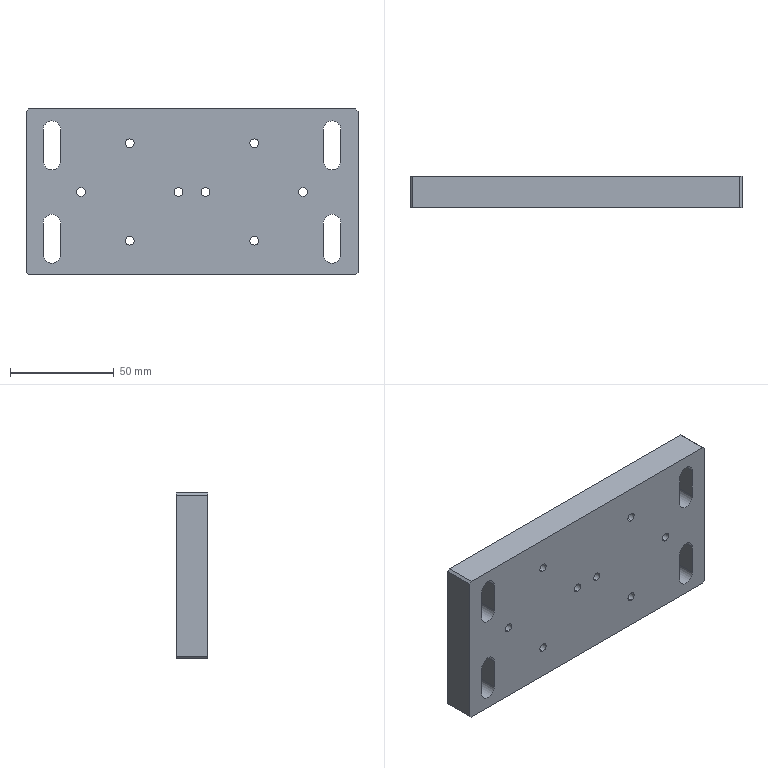Component | SolidWorks | CCDJSBottomFixingPlate-1 | 1 solid | 46 faces | box 160 x 15 x 80 mm | volume 179253 mm3 | cylinder 28 | plane 18 | commonest cylinder face diameters 4.2 x16 8.5 x12 | material 45#
build123d program:
from build123d import *

# Parameters (mm, degrees)
SKETCH1_W           = 160
SKETCH1_H           = 80
BOSS_EXTRUDE1_DEPTH = 15
CHAMFER1_SIZE       = 1
CUT_EXTRUDE1_DEPTH  = 32
M5_TAPPED_HOLE1_D   = 4.2


with BuildPart() as part:
    # Sketch1 → Boss-Extrude1 (new body)
    with BuildSketch(Plane(origin=(0, 0, 0), x_dir=(1, 0, 0), z_dir=(0, 1, 0))):
        Rectangle(SKETCH1_W, SKETCH1_H)
    extrude(amount=BOSS_EXTRUDE1_DEPTH)

    # Chamfer1
    chamfer1_edges = [part.edges().sort_by_distance(p)[0] for p in [
        (80, 7.5, 40),
        (-80, 7.5, 40),
        (-80, 7.5, -40),
        (80, 7.5, -40),
    ]]
    chamfer(chamfer1_edges, length=CHAMFER1_SIZE)

    # Sketch2 → Cut-Extrude1 (cut)
    with BuildSketch(Plane(origin=(0, 15, 0), x_dir=(1, 0, 0), z_dir=(0, 1, 0))):
        with BuildLine():
            Line((-63.25, 30), (-63.25, 15))
            ThreePointArc((-63.25, 15), (-67.5, 10.75), (-71.75, 15))
            Line((-71.75, 15), (-71.75, 30))
            ThreePointArc((-71.75, 30), (-67.5, 34.25), (-63.25, 30))
        make_face()
        with BuildLine():
            Line((-63.25, -30), (-63.25, -15))
            ThreePointArc((-63.25, -15), (-67.5, -10.75), (-71.75, -15))
            Line((-71.75, -15), (-71.75, -30))
            ThreePointArc((-71.75, -30), (-67.5, -34.25), (-63.25, -30))
        make_face()
        with BuildLine():
            Line((63.25, -30), (63.25, -15))
            ThreePointArc((63.25, -15), (67.5, -10.75), (71.75, -15))
            Line((71.75, -15), (71.75, -30))
            ThreePointArc((71.75, -30), (67.5, -34.25), (63.25, -30))
        make_face()
        with BuildLine():
            Line((63.25, 30), (63.25, 15))
            ThreePointArc((63.25, 15), (67.5, 10.75), (71.75, 15))
            Line((71.75, 15), (71.75, 30))
            ThreePointArc((71.75, 30), (67.5, 34.25), (63.25, 30))
        make_face()
    extrude(amount=-CUT_EXTRUDE1_DEPTH, mode=Mode.SUBTRACT)

    # M5 Tapped Hole1 (through all)
    with Locations(Plane(origin=(0, 15, 0), x_dir=(1, 0, 0), z_dir=(0, 1, 0))):
        with Locations((-30, 23.5), (-6.5, 0), (-53.5, 0), (-30, -23.5), (30, -23.5), (53.5, 0), (6.5, 0), (30, 23.5)):
            Hole(M5_TAPPED_HOLE1_D / 2)


solid = part.part